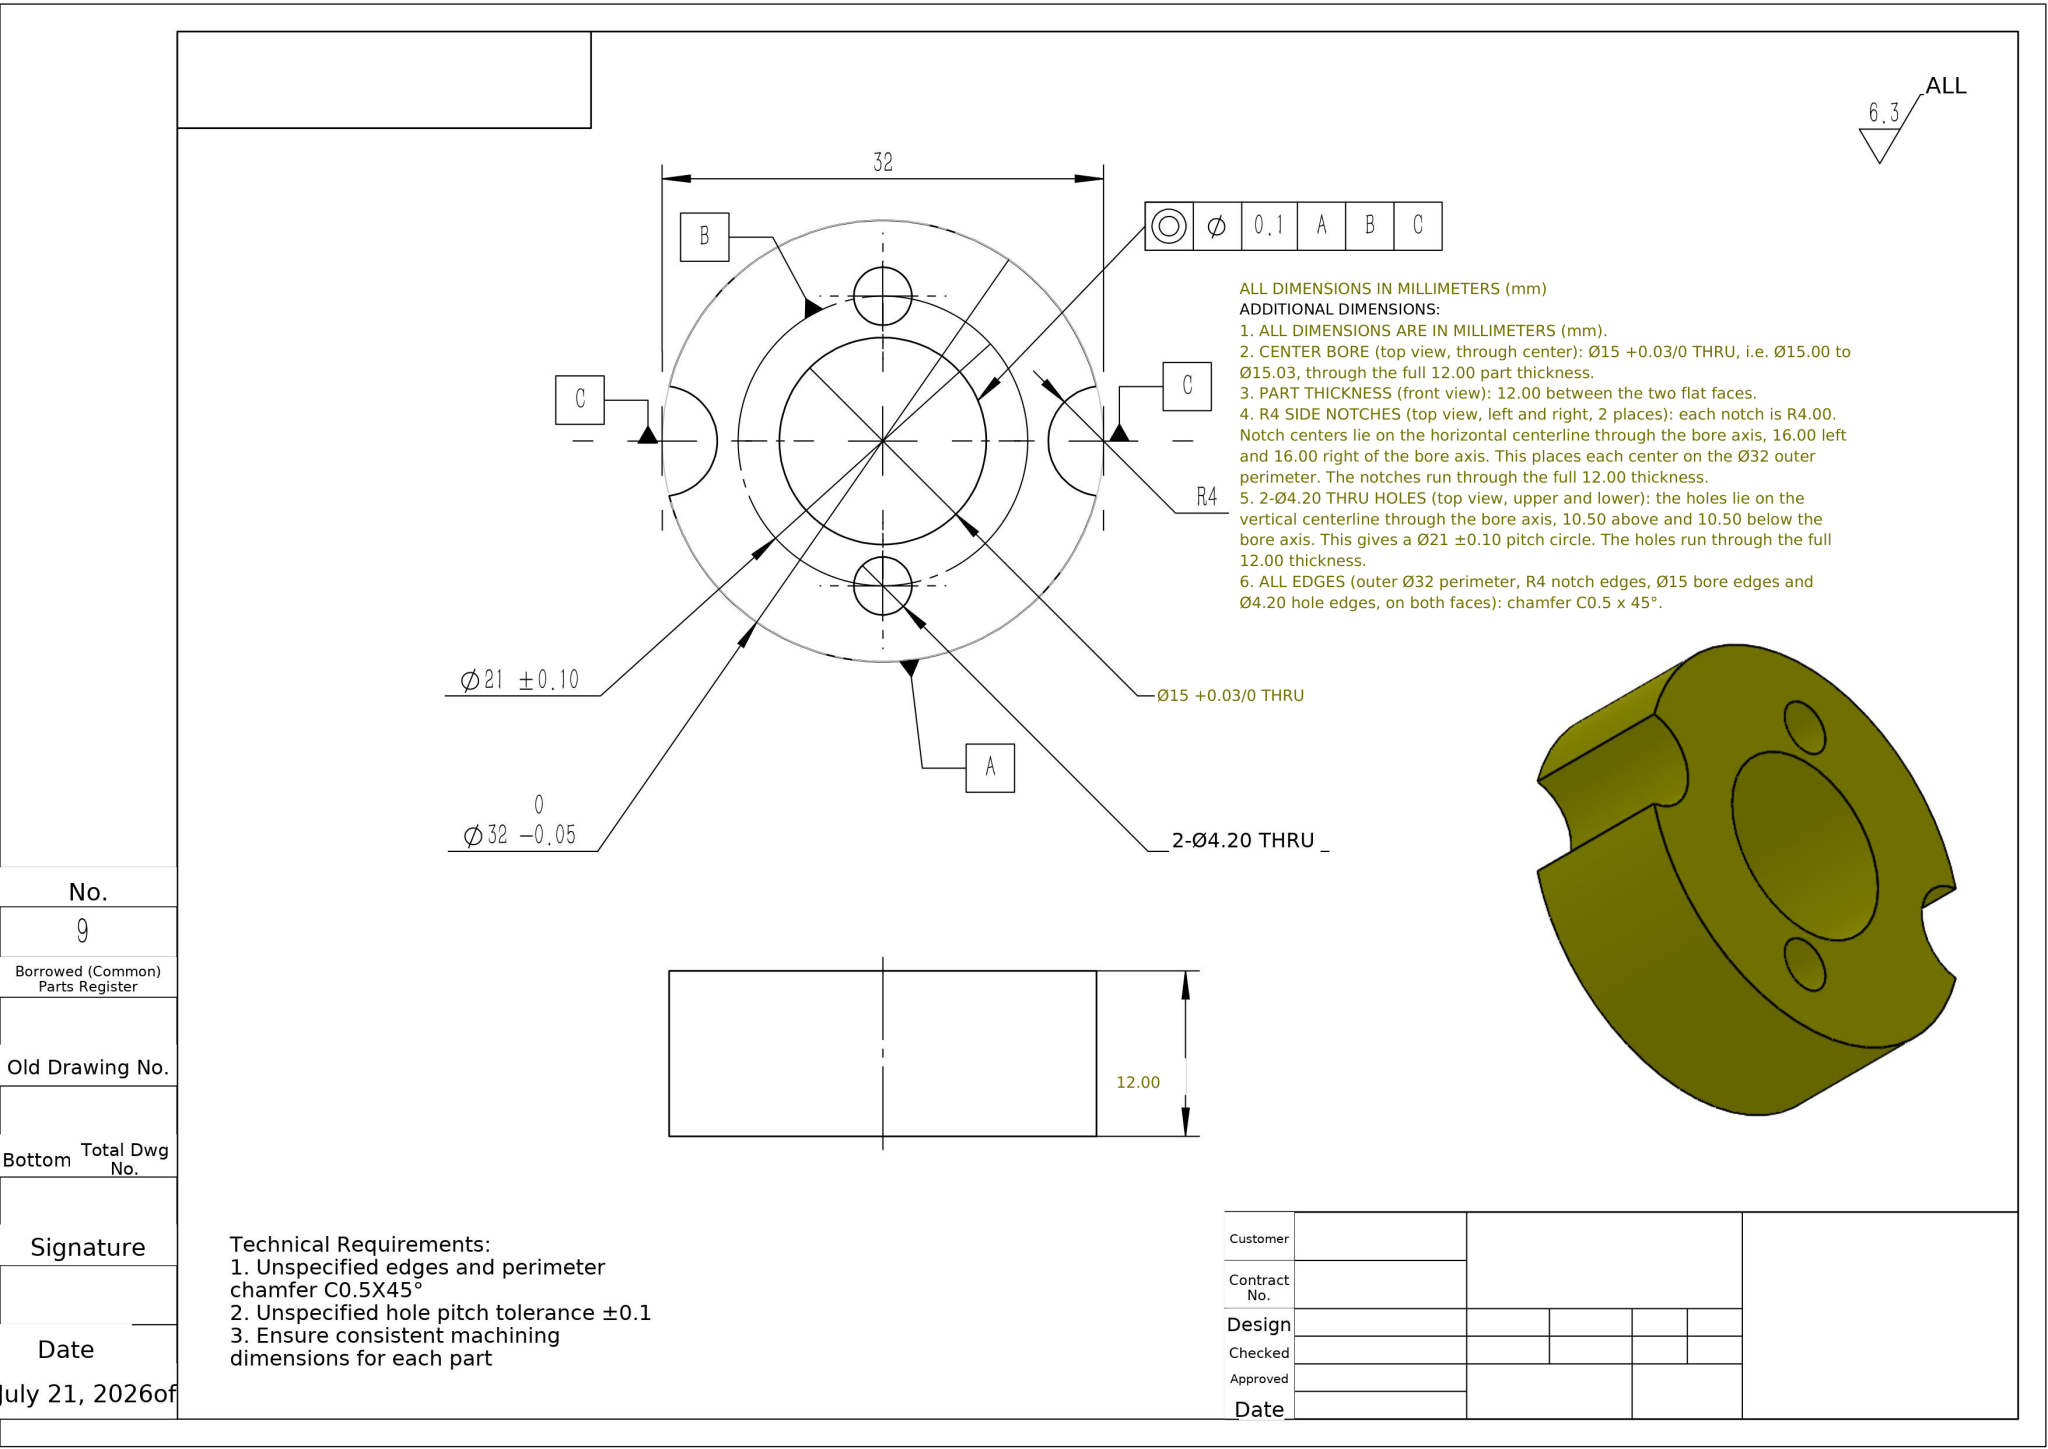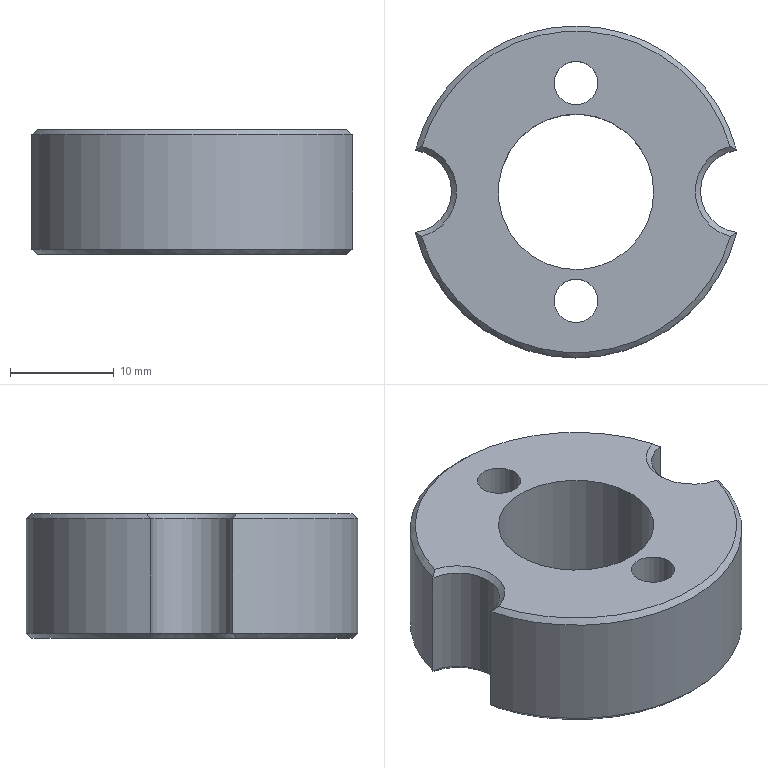Part | NX | mm | Notched Flanged Drum Mount | 1 solid | 17 faces | box 31.03 x 32 x 12 mm | volume 6600 mm3 | cone 8 | cylinder 7 | plane 2 | commonest cylinder face diameters 32 x2 8 x2 4.2 x2 15 x1